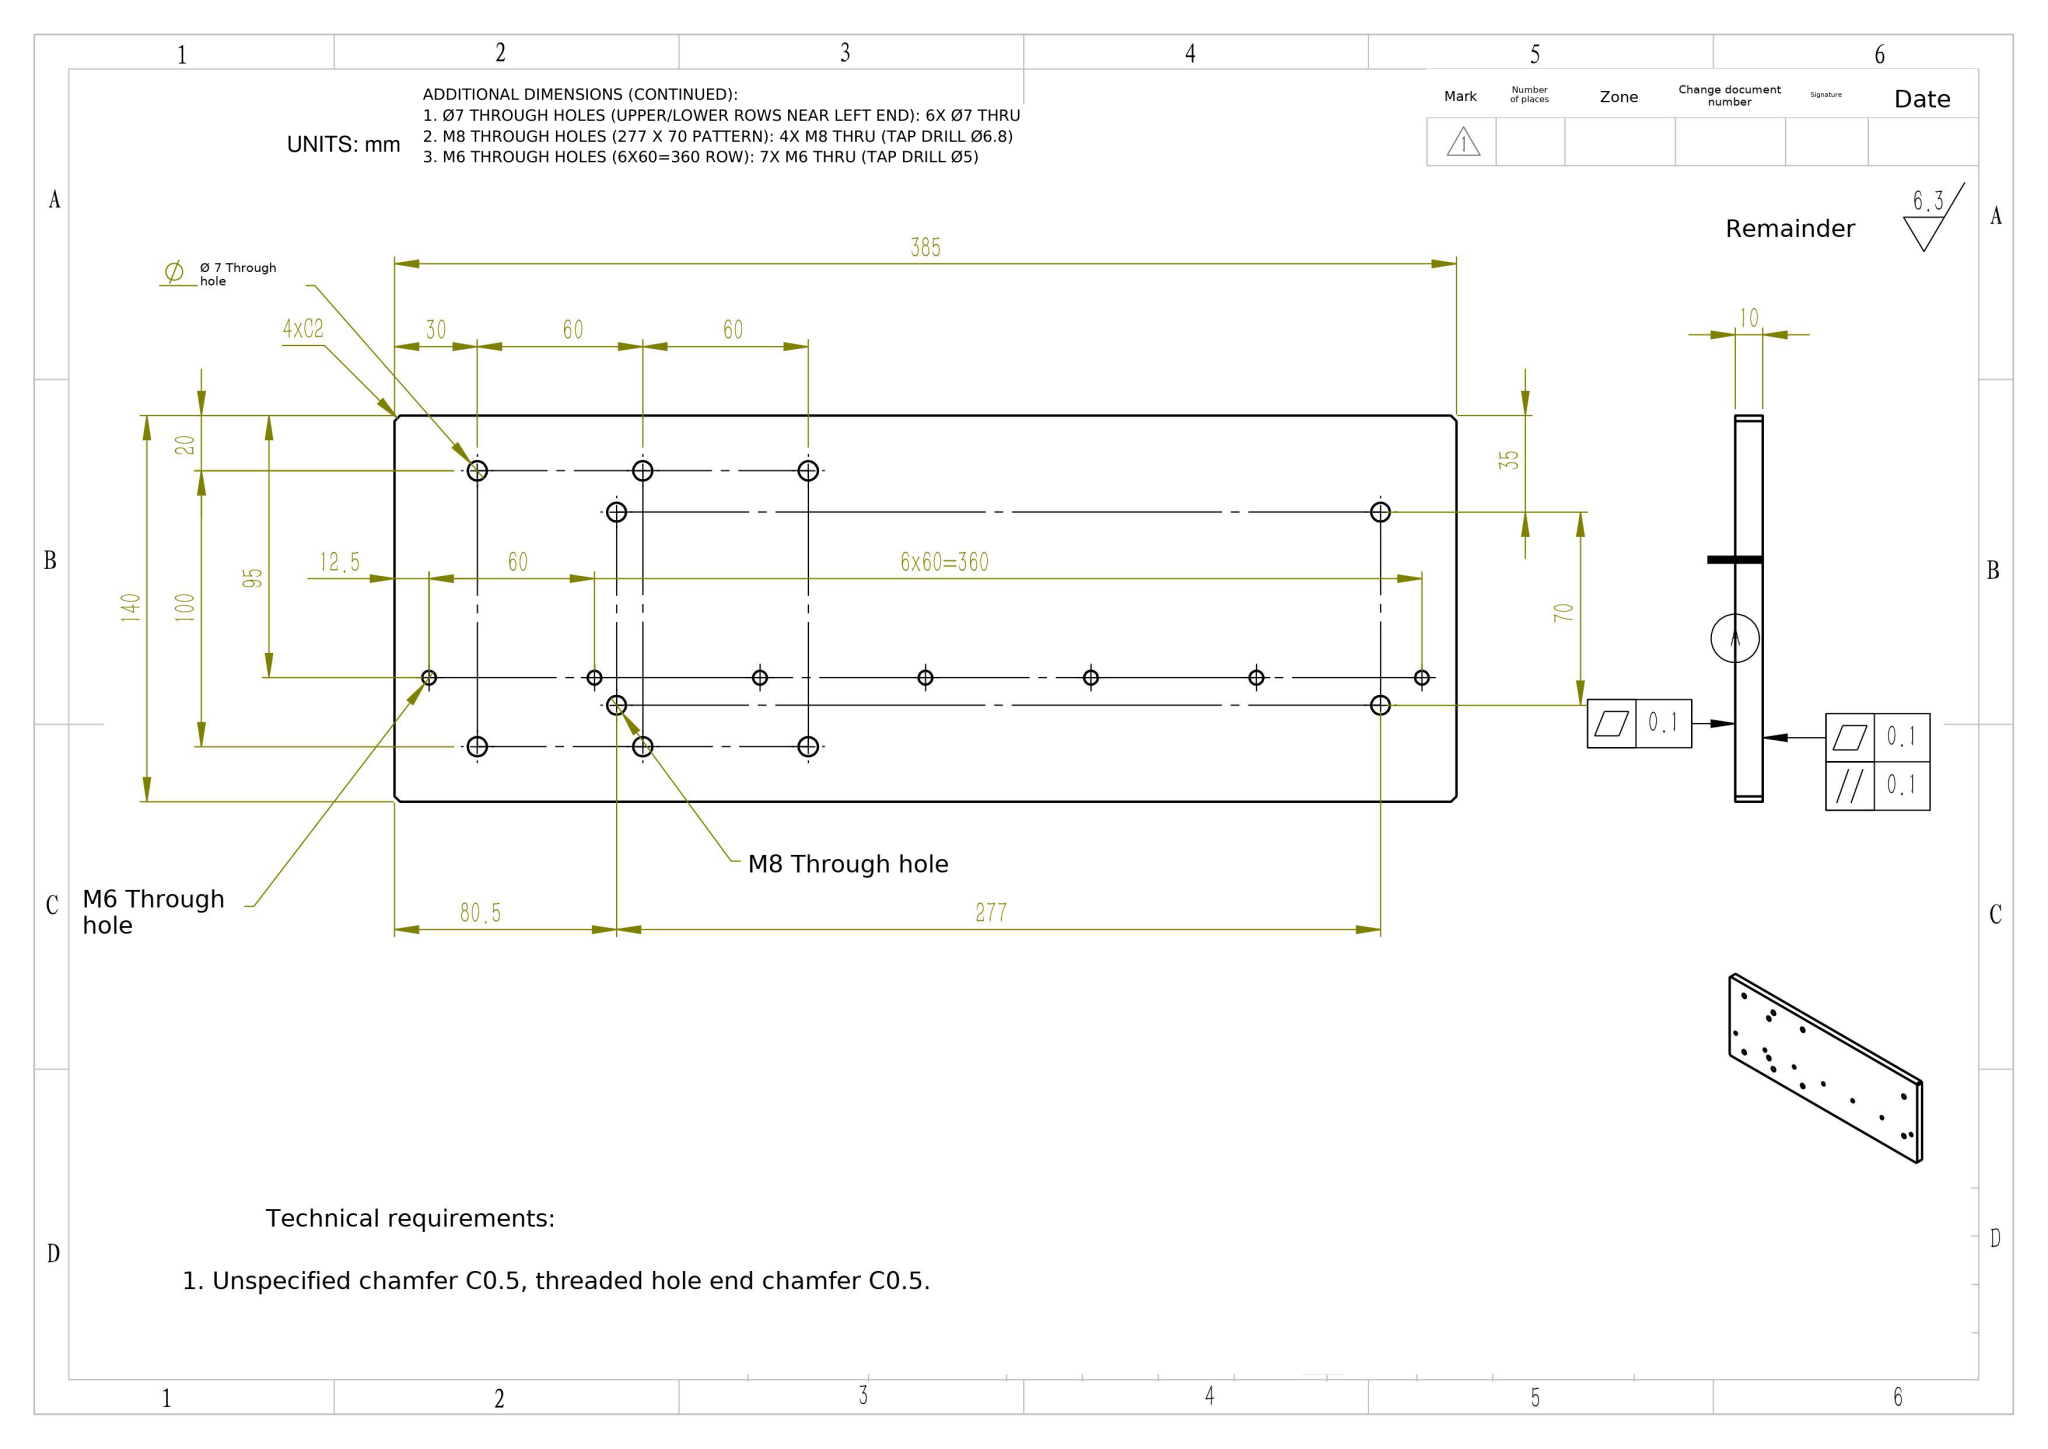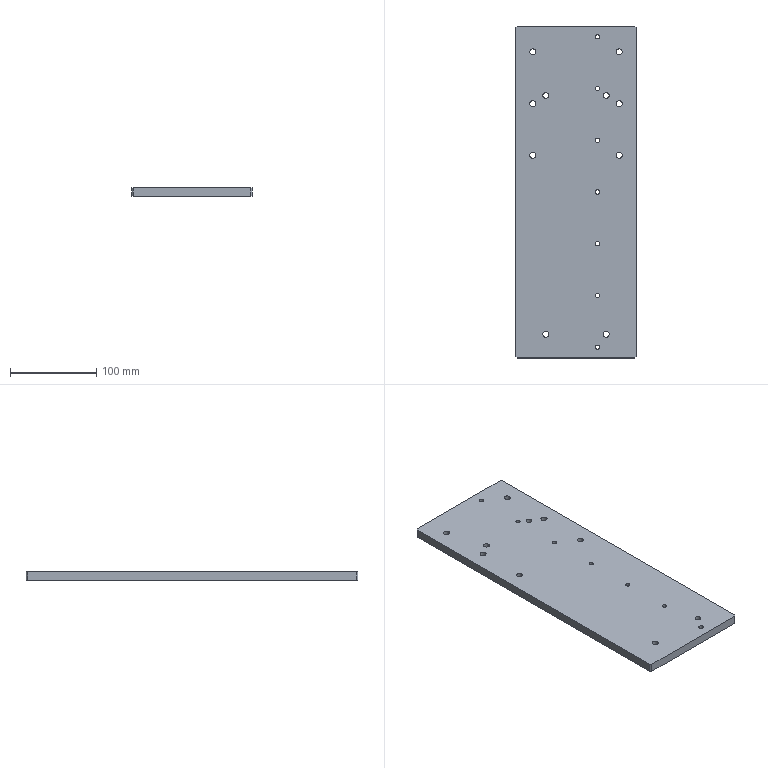Part | NX | mm | 1 solid | 44 faces | box 140 x 385 x 10 mm | volume 533784 mm3 | cylinder 34 | plane 10 | commonest cylinder face diameters 5 x14 7 x12 6.8 x8